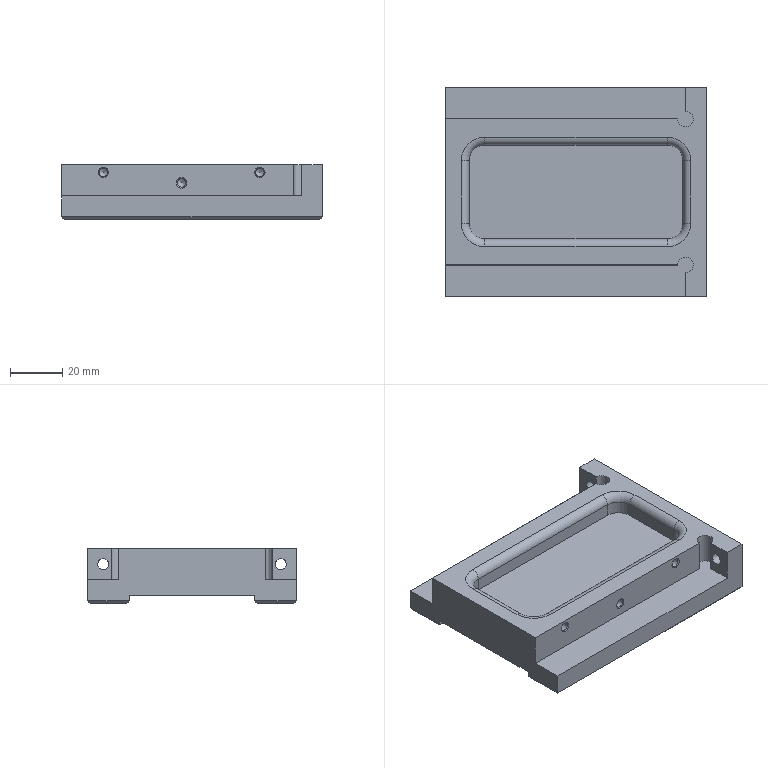Component | NX | BASE | 1 solid | 67 faces | volume 101592 mm3 | plane 31 | cylinder 20 | cone 12 | torus 4 | commonest cylinder face diameters 6 x6 3.3 x6 12 x4 4.3 x2 7.5 x2